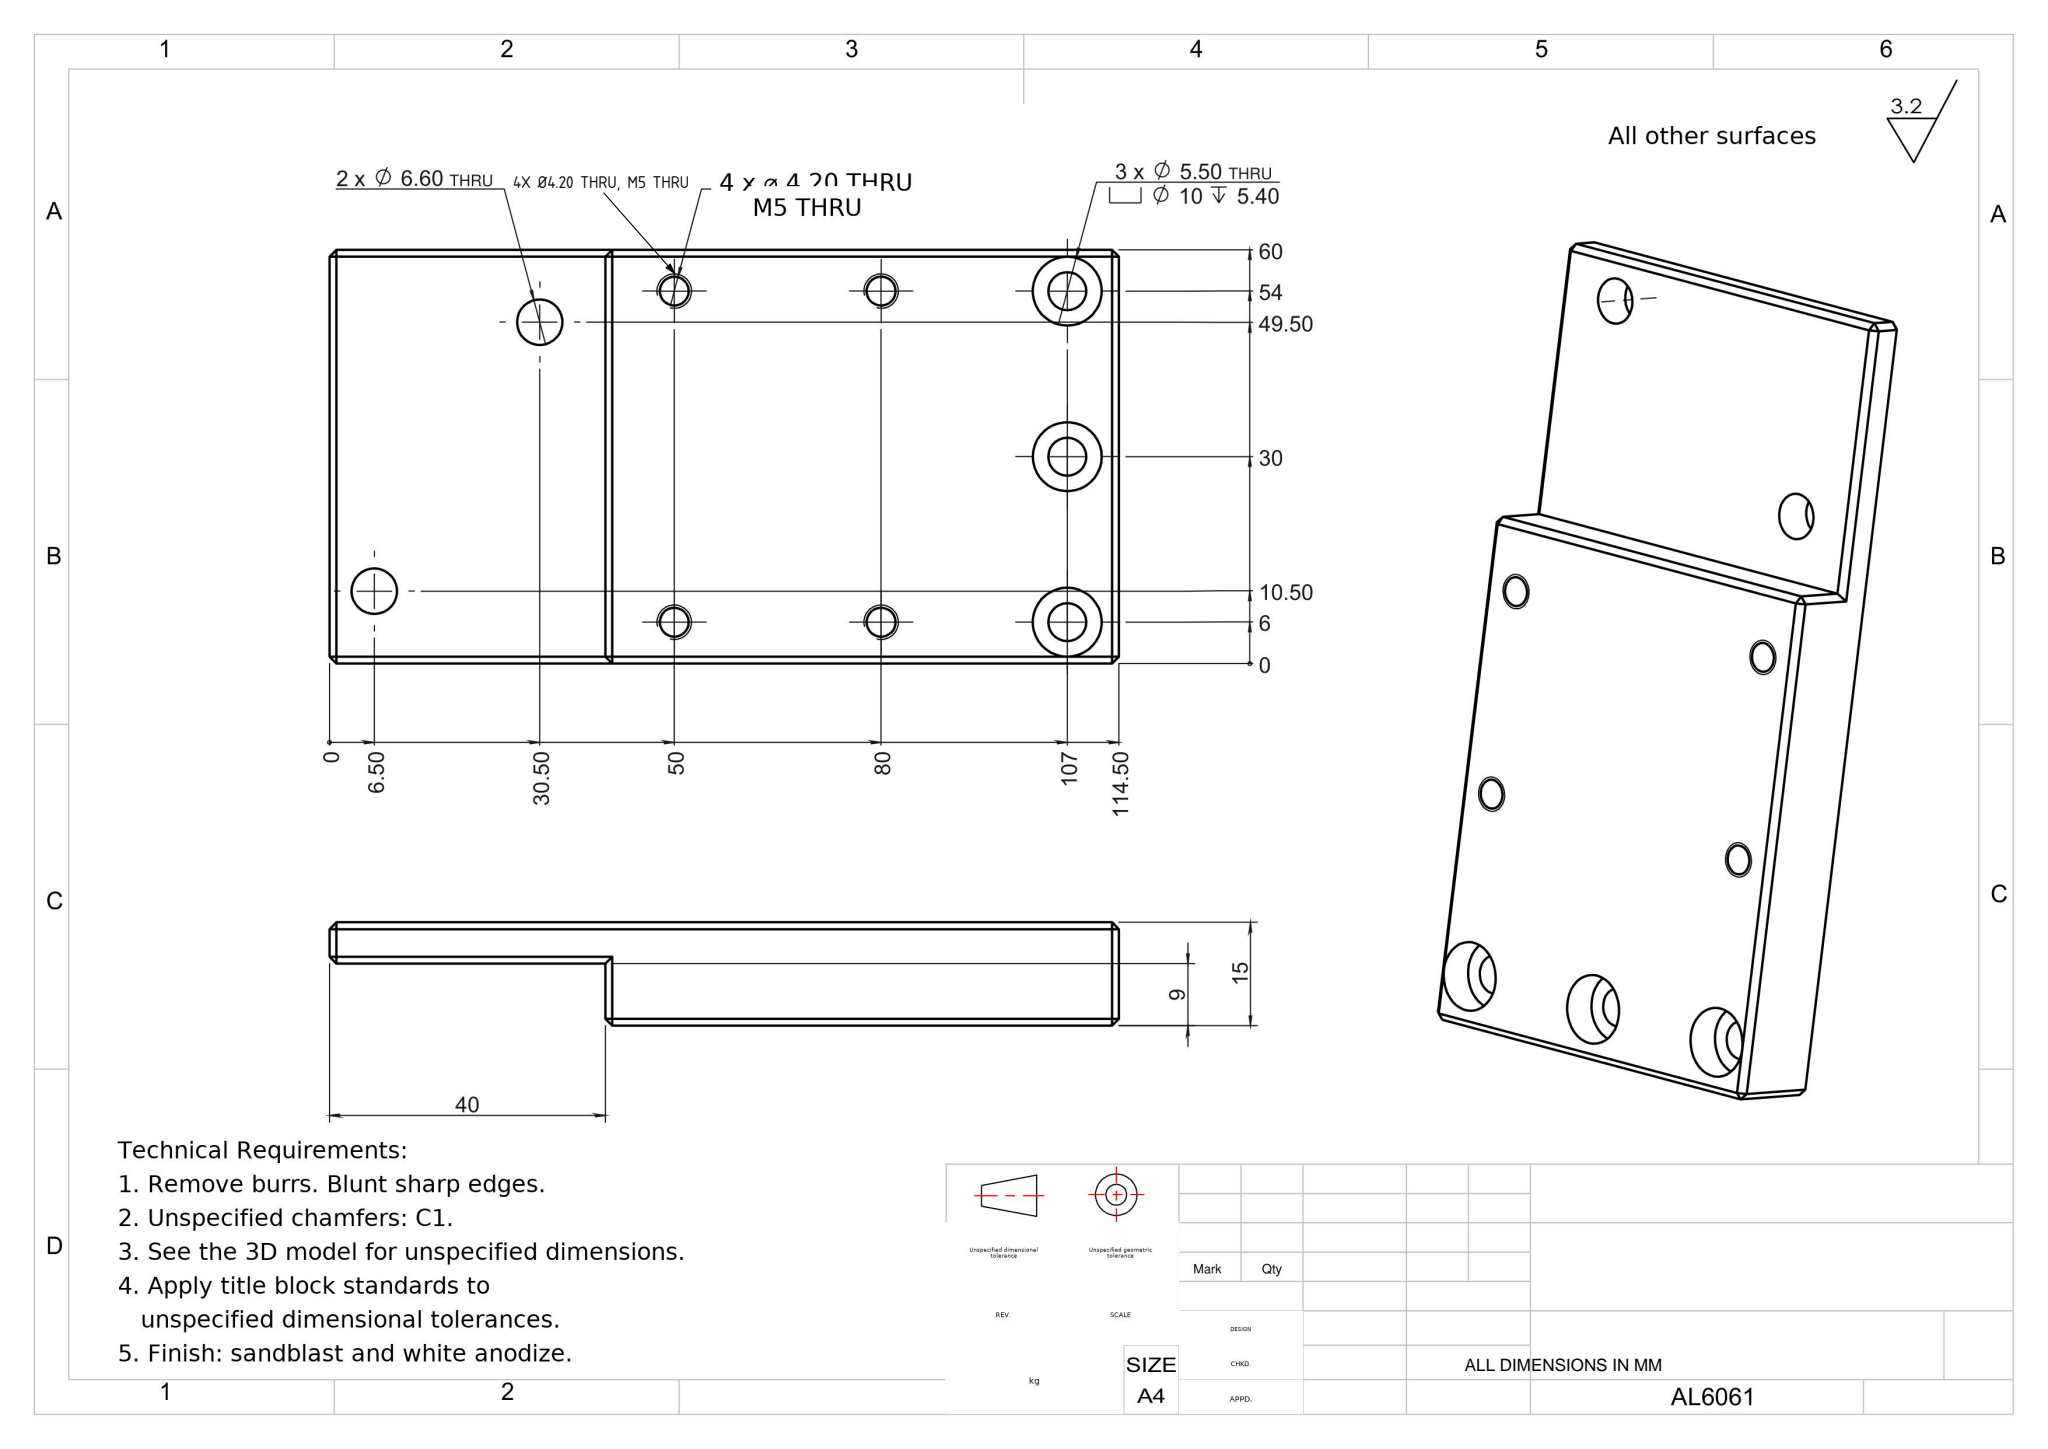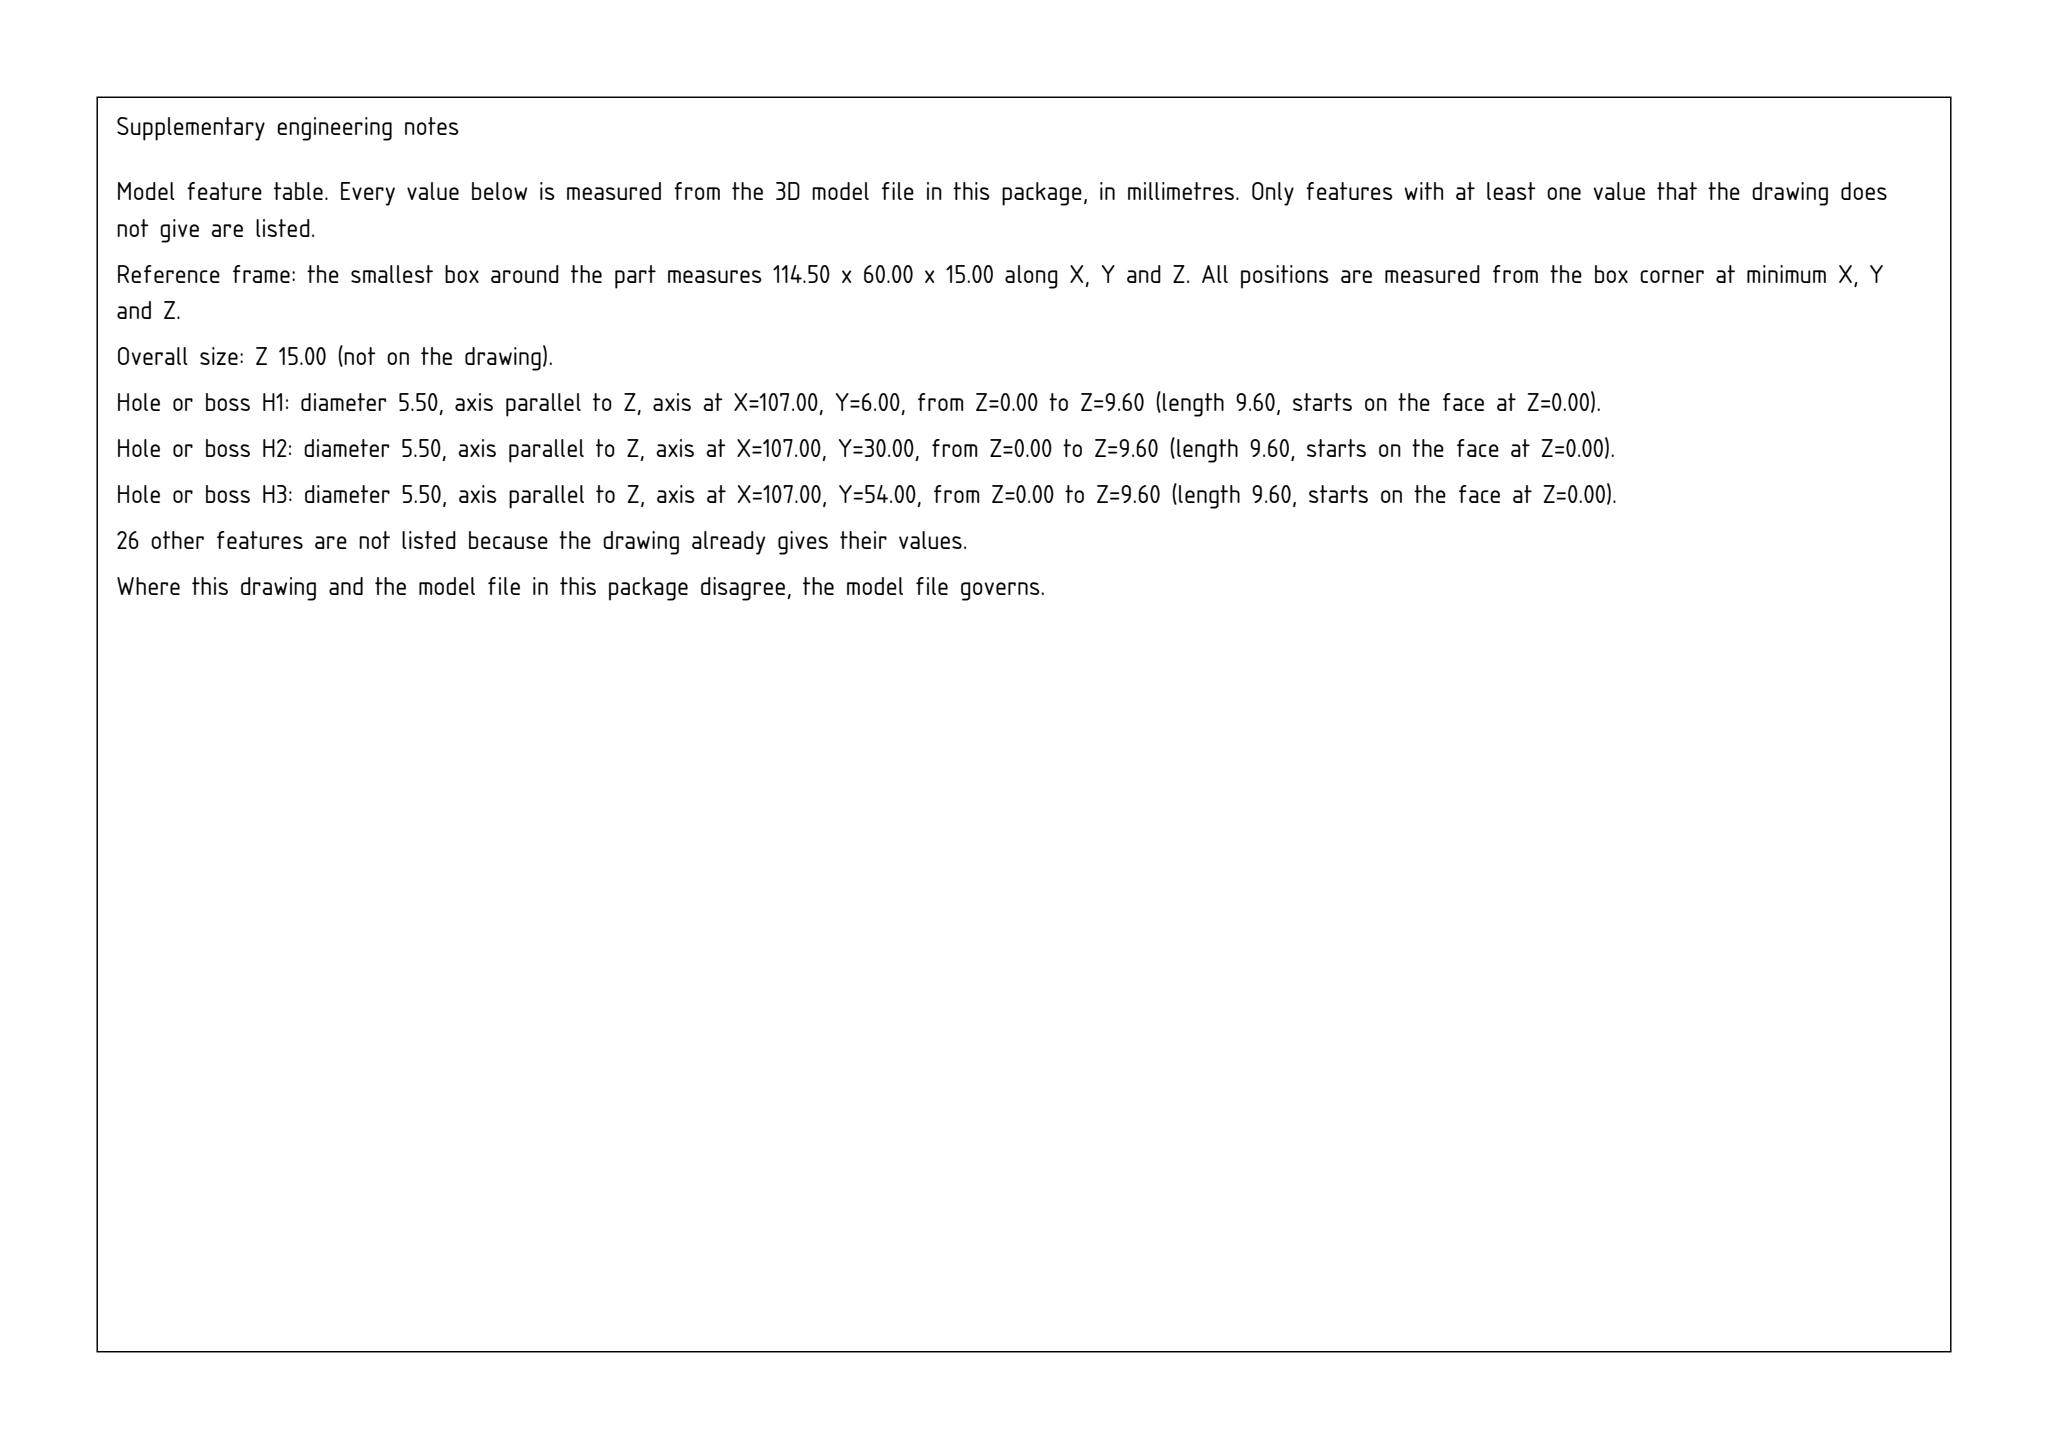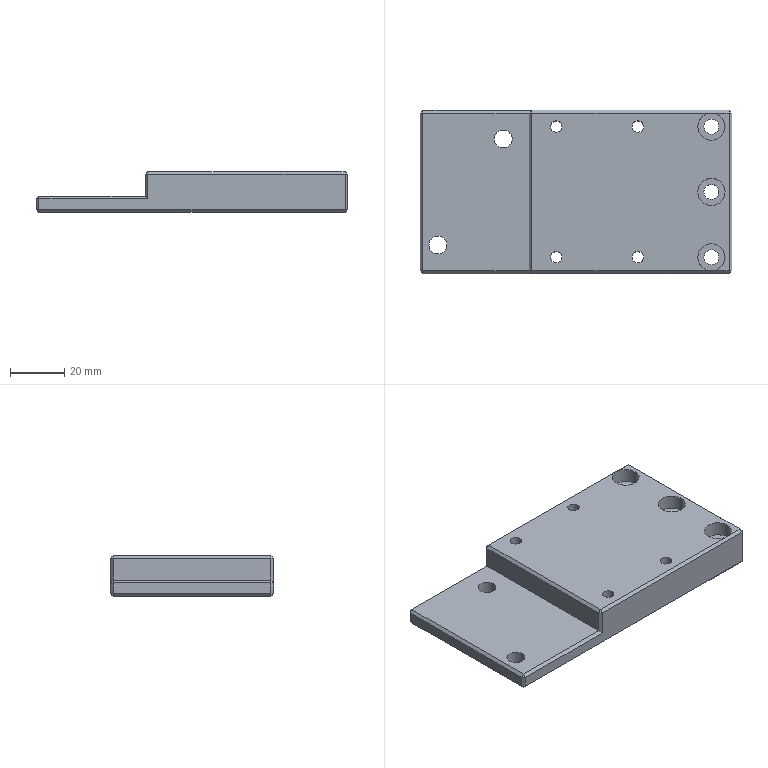Part | SolidWorks | mm | material AL6061 | 1 solid | 62 faces | box 114.5 x 60 x 15 mm | volume 77849 mm3 | plane 38 | cylinder 24 | commonest cylinder face diameters 4.2 x8 10 x6 5.5 x6 6.6 x4
Drawing notes:
4 x Ø4.20 THRU, M5 THRU | from the solid: Four Ø4.2 z-axis thru holes at (50,54),(50,6),(80,54),(80,6), z 0-15